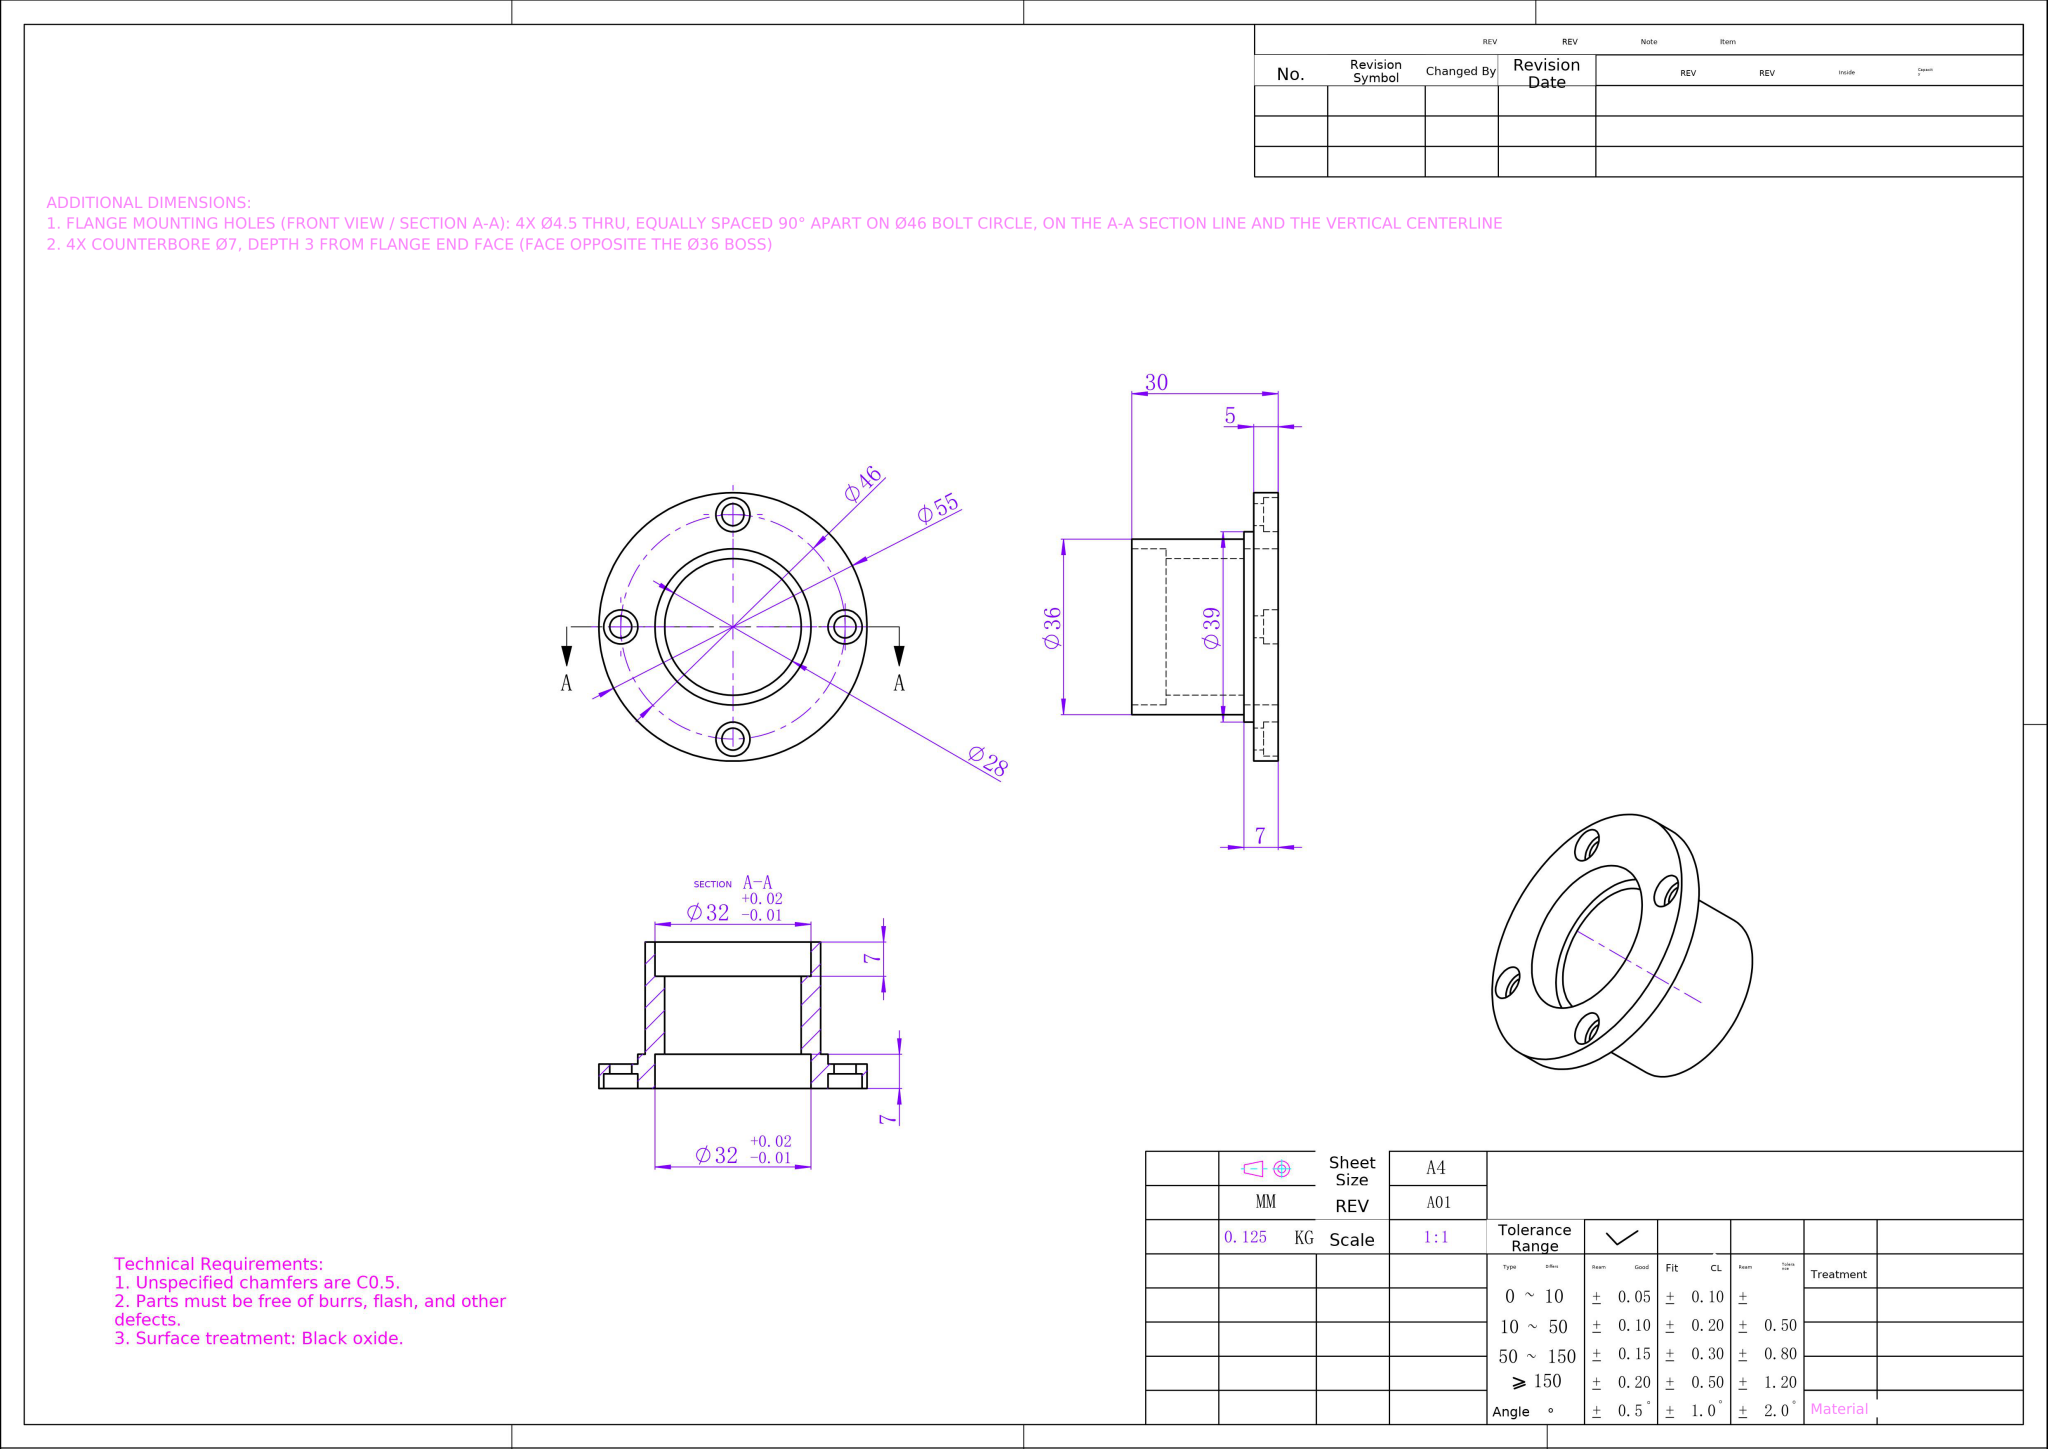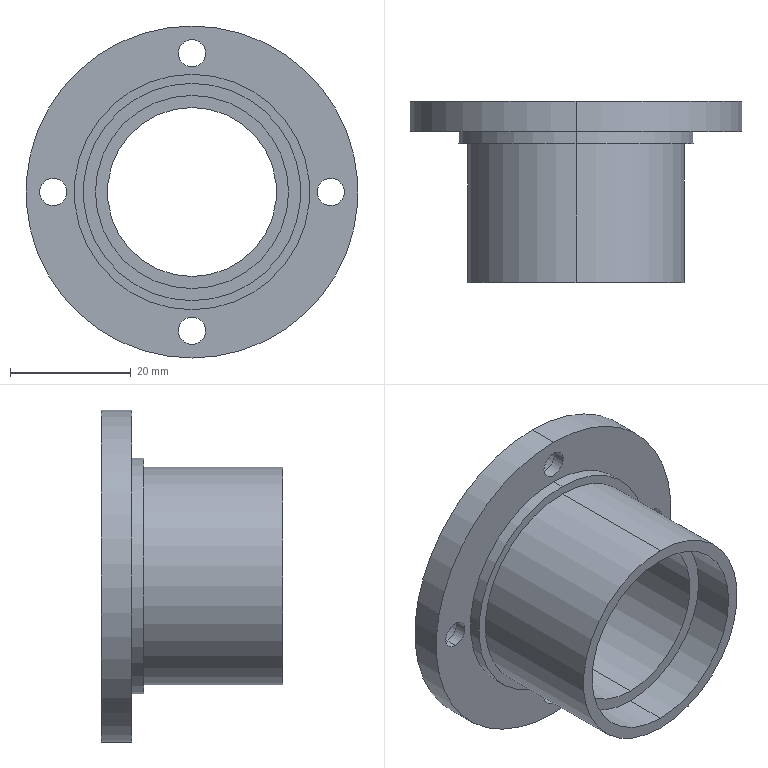Part | NX | mm | 1 solid | 38 faces | box 55 x 30 x 55 mm | volume 15979 mm3 | cylinder 28 | plane 10 | commonest cylinder face diameters 7 x8 4.5 x8 32 x4 39 x2 28 x2 55 x2 36 x2